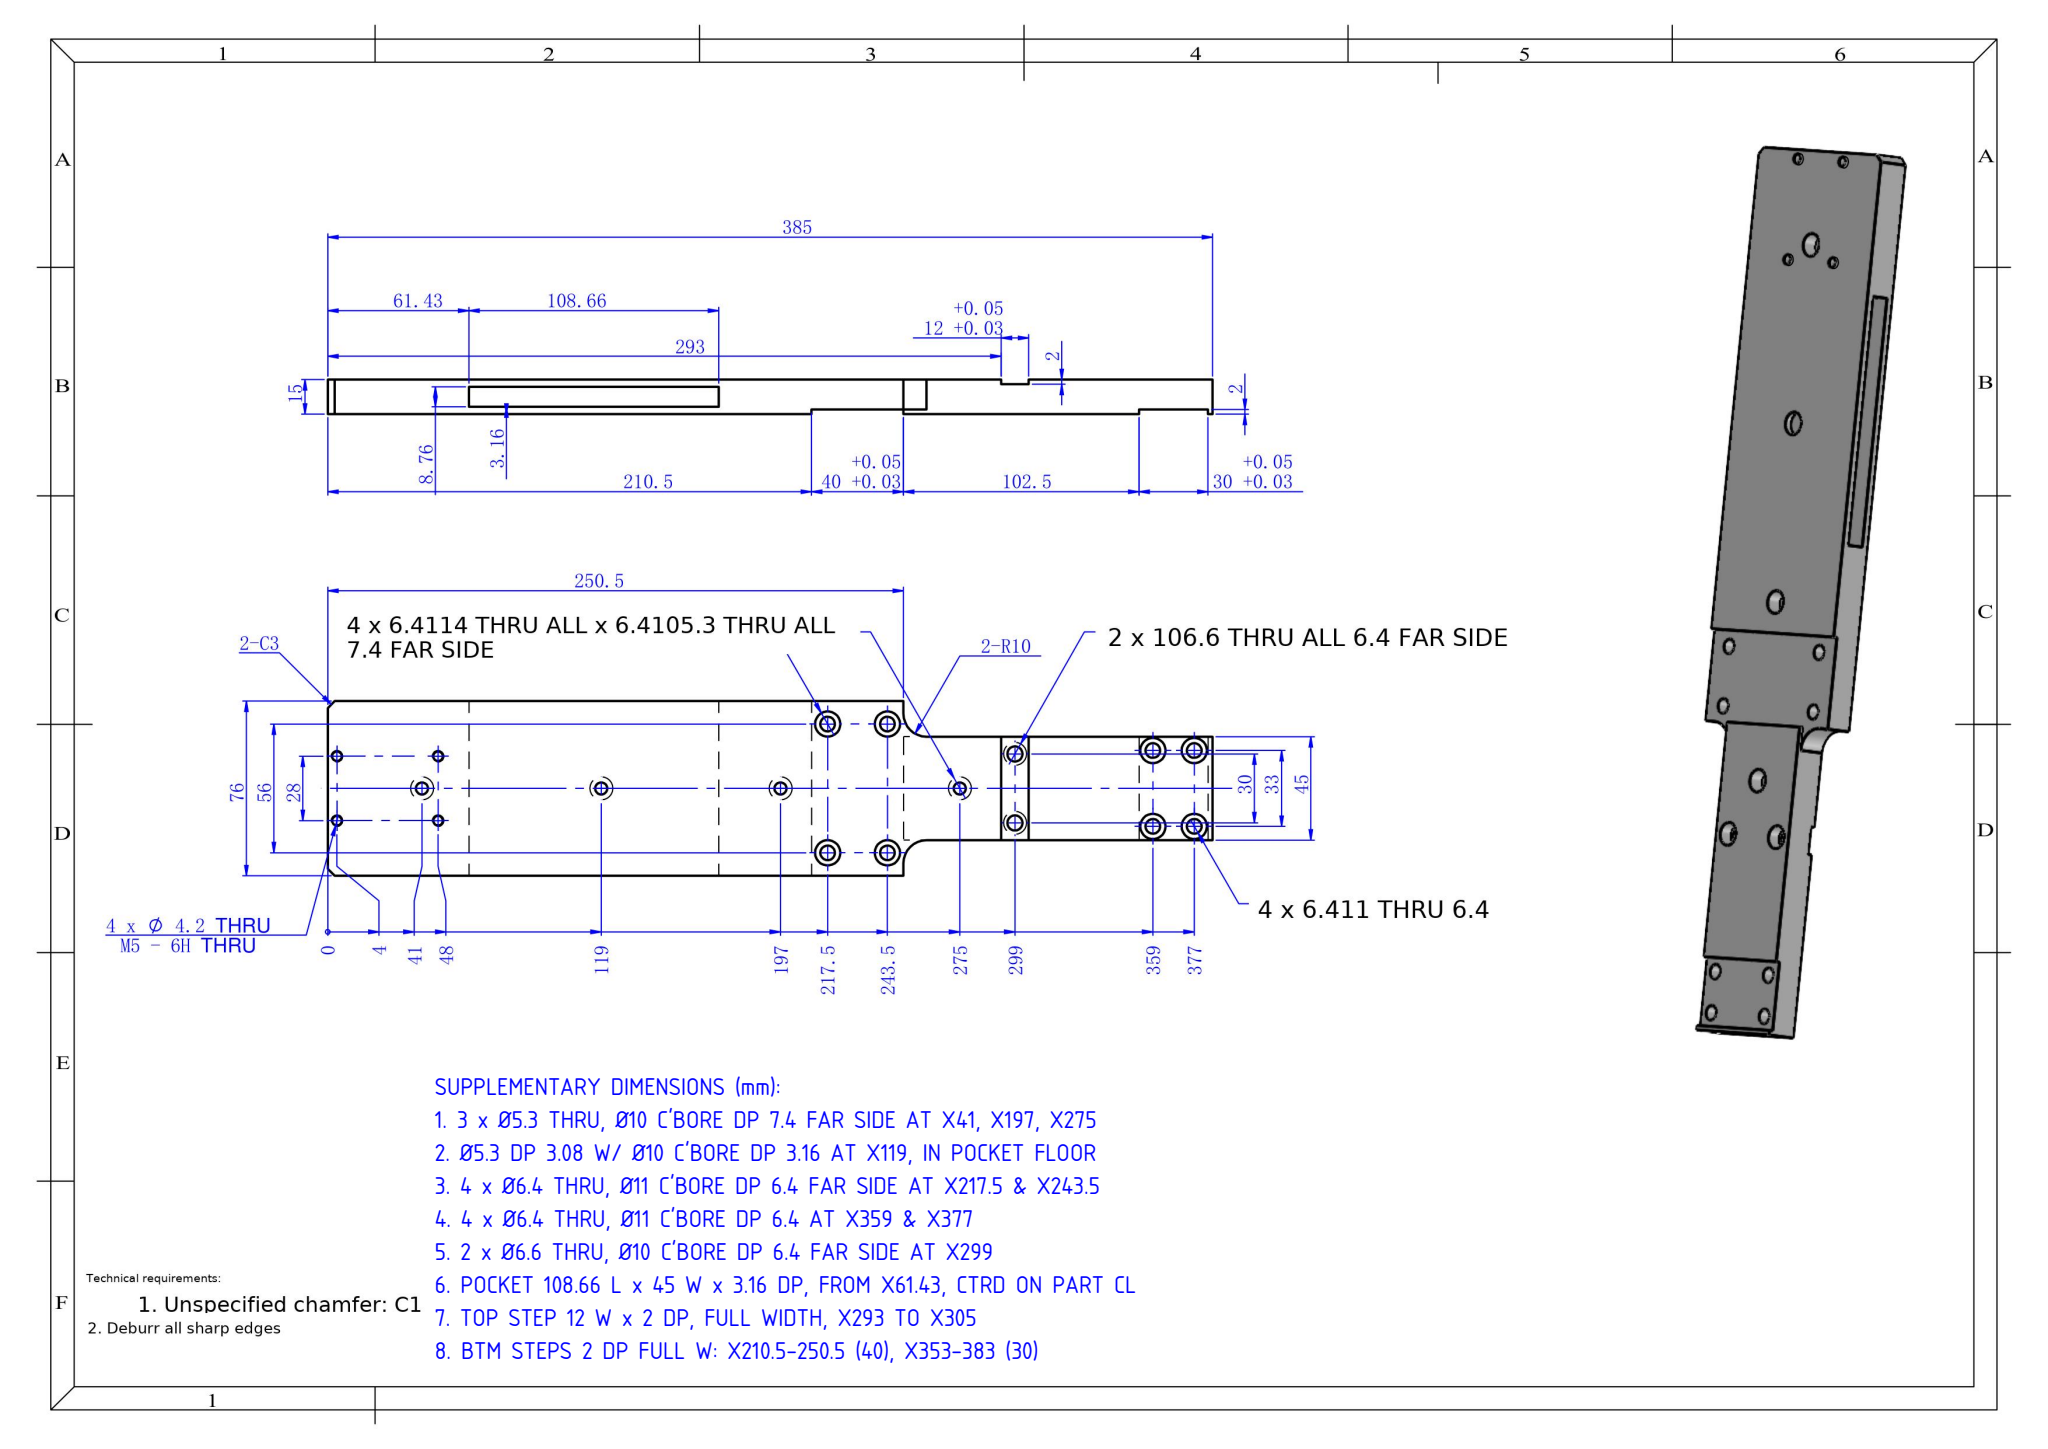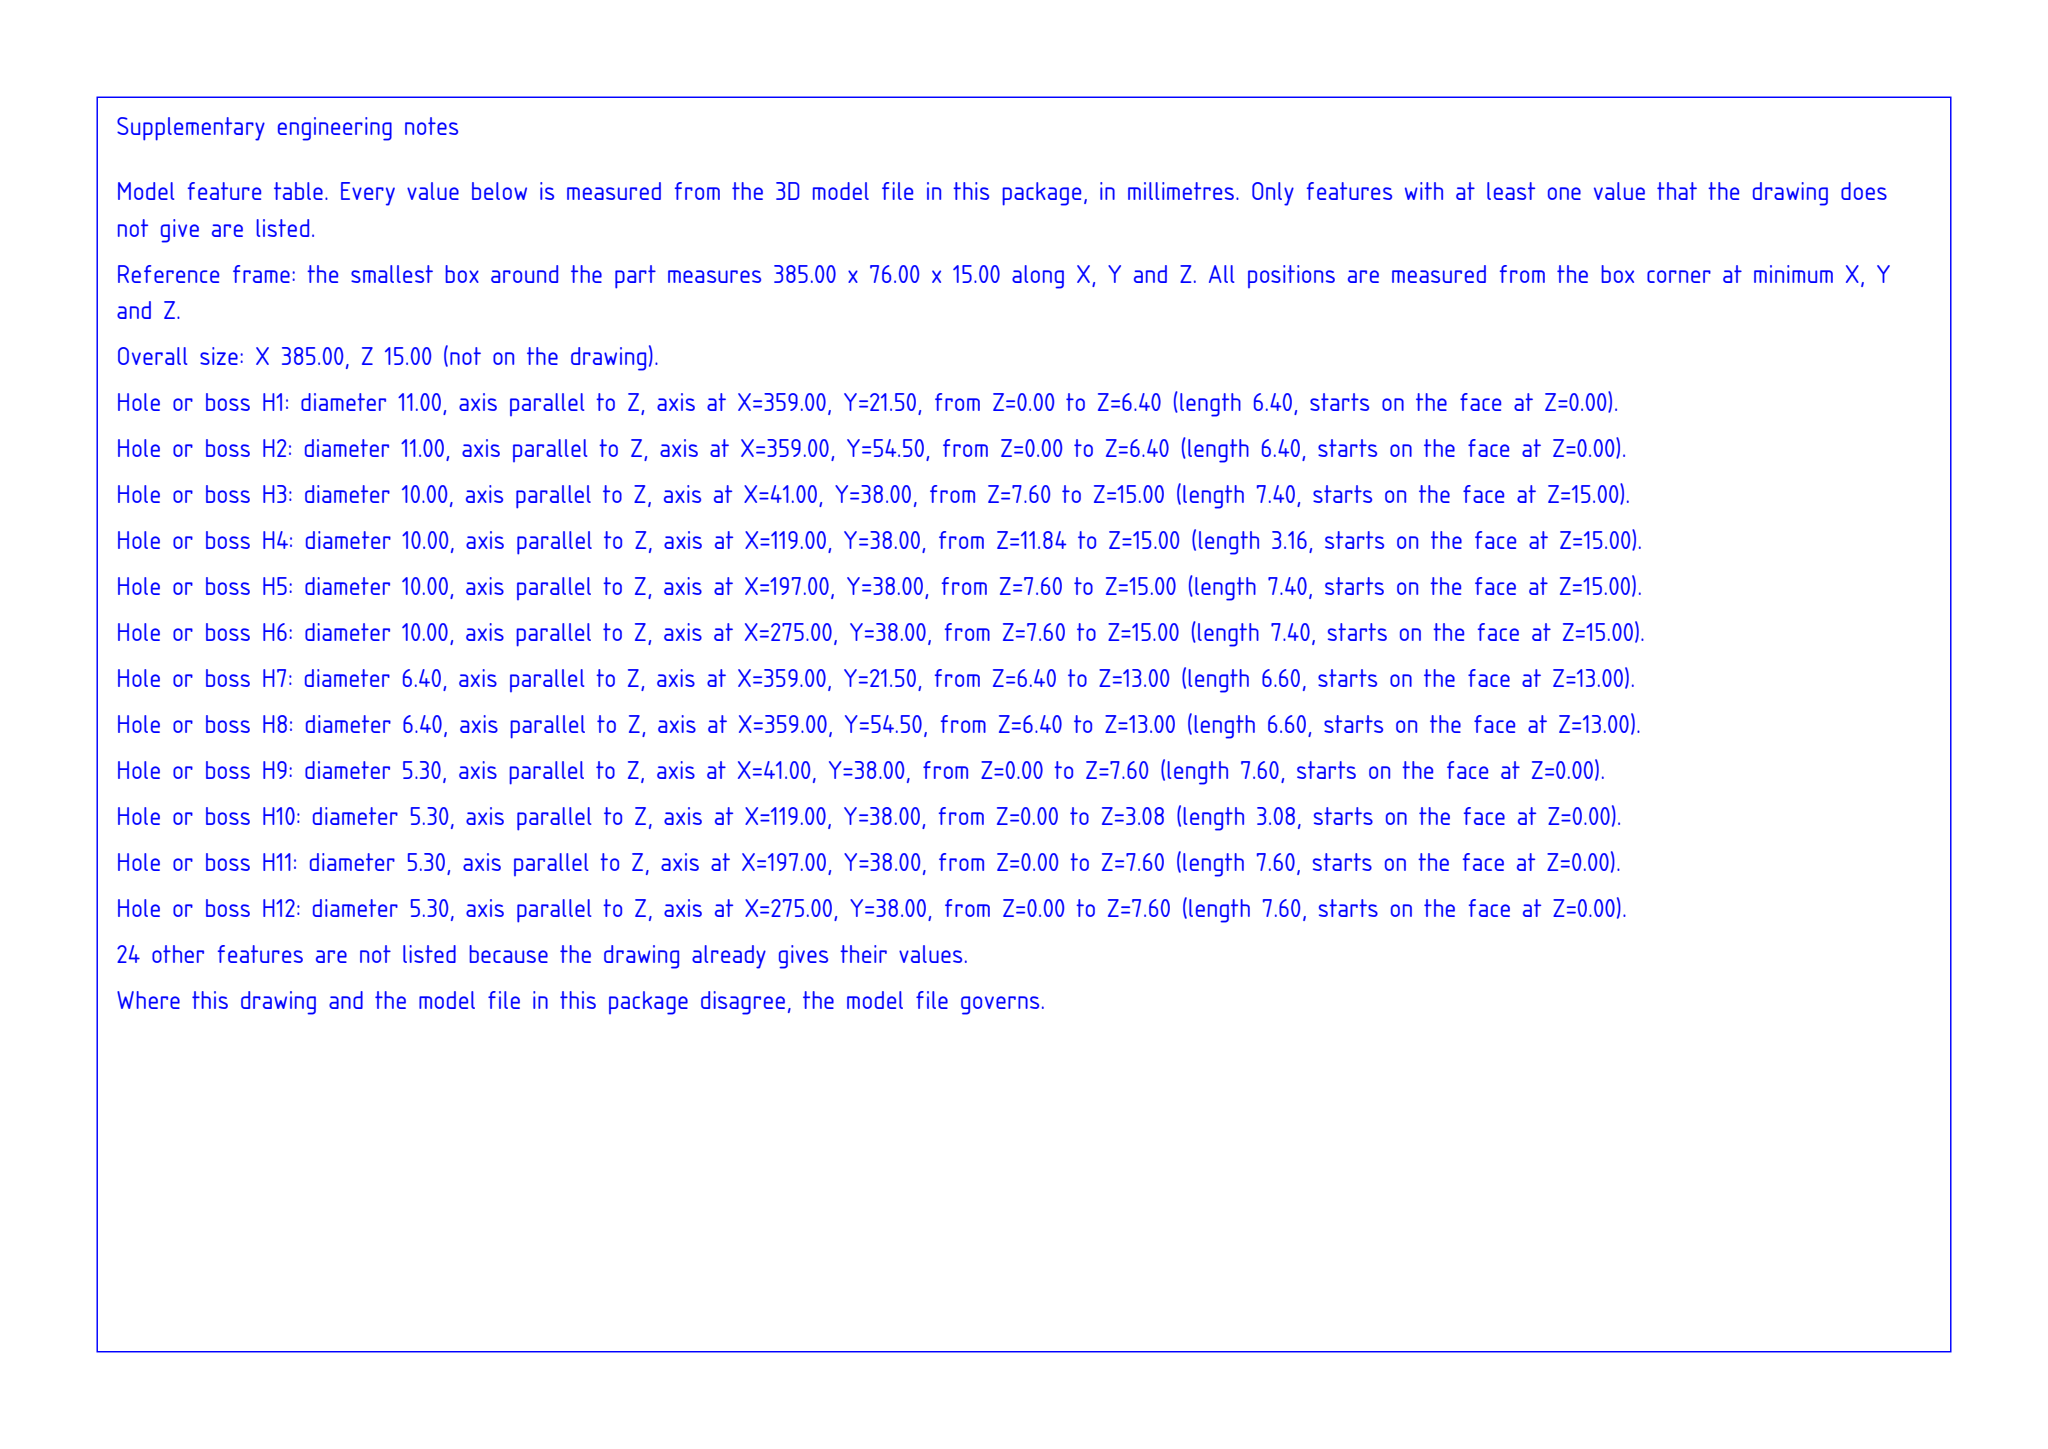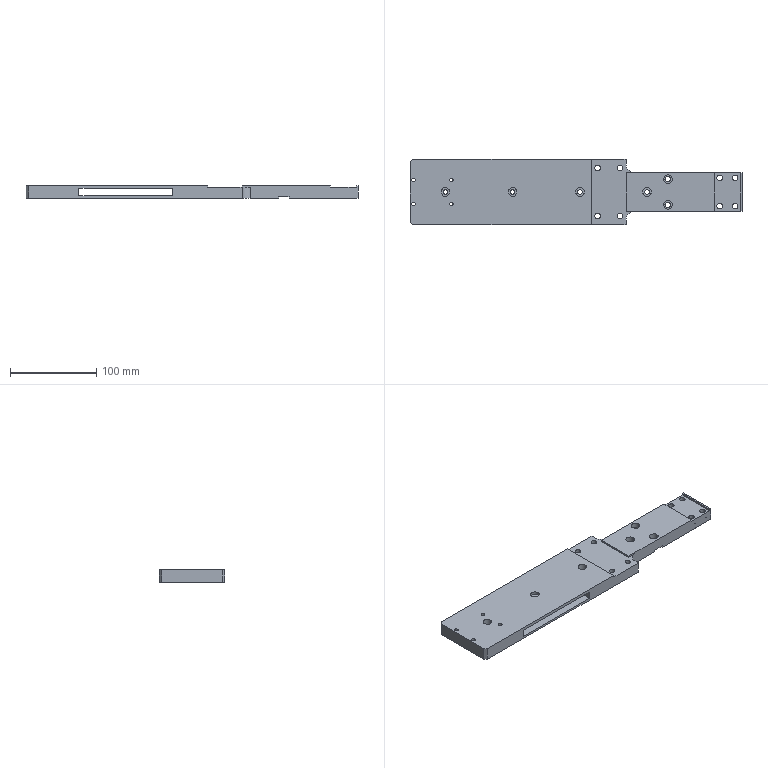Part | SolidWorks | mm | 1 solid | 107 faces | box 385 x 76 x 15 mm | volume 283123 mm3 | cylinder 66 | plane 41 | commonest cylinder face diameters 11 x16 6.4 x16 10 x12 4.2 x8 5.3 x8 6.6 x4 20 x2
build123d program:
from build123d import *

# Parameters (mm, degrees)
SKETCH1_W                                       = 385
SKETCH1_H                                       = 76
BOSS_EXTRUDE1_DEPTH                             = 15
SKETCH10_W                                      = 30
SKETCH10_H                                      = 2
SKETCH10_W_2                                    = 40
CUT_EXTRUDE5_DEPTH                              = 320.688
SKETCH12_W                                      = 134.5
SKETCH12_H                                      = 15.5
CUT_EXTRUDE10_DEPTH                             = 317.416
FILLET1_R                                       = 10
M6_HEX_SOCKET_HEAD_CAP_SCREW_CBORE1_D           = 6.4
M6_HEX_SOCKET_HEAD_CAP_SCREW_CBORE1_CBORE_D     = 11
M6_HEX_SOCKET_HEAD_CAP_SCREW_CBORE1_CBORE_DEPTH = 6.4
M6_HEX_SOCKET_HEAD_CAP_SCREW_CBORE2_D           = 6.4
M6_HEX_SOCKET_HEAD_CAP_SCREW_CBORE2_CBORE_D     = 11
M6_HEX_SOCKET_HEAD_CAP_SCREW_CBORE2_CBORE_DEPTH = 6.4
SKETCH17_W                                      = 12
SKETCH17_H                                      = 2
CUT_EXTRUDE11_DEPTH                             = 317.362
M5_HEX_SOCKET_HEAD_CAP_SCREW_CBORE1_D           = 5.3
M5_HEX_SOCKET_HEAD_CAP_SCREW_CBORE1_CBORE_D     = 10
M5_HEX_SOCKET_HEAD_CAP_SCREW_CBORE1_CBORE_DEPTH = 7.4
M5_TAPPED_HOLE1_D                               = 4.2
M6_HEX_SOCKET_HEAD_CAP_SCREW_CBORE3_D           = 6.6
M6_HEX_SOCKET_HEAD_CAP_SCREW_CBORE3_CBORE_D     = 10
M6_HEX_SOCKET_HEAD_CAP_SCREW_CBORE3_CBORE_DEPTH = 6.4
CHAMFER1_SIZE                                   = 3
SKETCH28_W                                      = 108.663
SKETCH28_H                                      = 8.765
CUT_EXTRUDE12_DEPTH                             = 133


with BuildPart() as part:
    # Sketch1 → Boss-Extrude1 (new body)
    with BuildSketch(Plane.XY):
        with Locations((117.661, 22.784)):
            Rectangle(SKETCH1_W, SKETCH1_H)
    extrude(amount=BOSS_EXTRUDE1_DEPTH)

    # Sketch10 → Cut-Extrude5 (cut, through all)
    with BuildSketch(Plane(origin=(0, 60.784, 0), x_dir=(1, 0, 0), z_dir=(0, 1, 0))):
        with Locations((293.161, -14)):
            Rectangle(SKETCH10_W, SKETCH10_H)
        with Locations((155.661, -14)):
            Rectangle(SKETCH10_W_2, SKETCH10_H)
    extrude(amount=-CUT_EXTRUDE5_DEPTH, mode=Mode.SUBTRACT)

    # Sketch12 → Cut-Extrude10 (cut, through all)
    with BuildSketch(Plane.XY.offset(15)):
        with Locations((242.911, 53.034)):
            Rectangle(SKETCH12_W, SKETCH12_H)
        with Locations((242.911, -7.466)):
            Rectangle(SKETCH12_W, SKETCH12_H)
    extrude(amount=-CUT_EXTRUDE10_DEPTH, mode=Mode.SUBTRACT)

    # Fillet1
    fillet1_edges = [part.edges().sort_by_distance(p)[0] for p in [
        (175.661, 45.284, 6.5),
        (175.661, 0.2842, 6.5),
    ]]
    fillet(fillet1_edges, radius=FILLET1_R)

    # M6 Hex Socket Head Cap Screw CBORE1 (through all)
    with Locations(Plane(origin=(0, 0, 0), x_dir=(-1, 0, 0), z_dir=(0, 0, -1))):
        with Locations((-284.161, 39.284), (-284.161, 6.284), (-302.161, 6.284), (-302.161, 39.284)):
            CounterBoreHole(M6_HEX_SOCKET_HEAD_CAP_SCREW_CBORE1_D / 2, M6_HEX_SOCKET_HEAD_CAP_SCREW_CBORE1_CBORE_D / 2, M6_HEX_SOCKET_HEAD_CAP_SCREW_CBORE1_CBORE_DEPTH)

    # M6 Hex Socket Head Cap Screw CBORE2 (through all)
    with Locations(Plane(origin=(0, 0, 0), x_dir=(-1, 0, 0), z_dir=(0, 0, -1))):
        with Locations((-142.661, 50.784), (-142.661, -5.216), (-168.661, -5.216), (-168.661, 50.784)):
            CounterBoreHole(M6_HEX_SOCKET_HEAD_CAP_SCREW_CBORE2_D / 2, M6_HEX_SOCKET_HEAD_CAP_SCREW_CBORE2_CBORE_D / 2, M6_HEX_SOCKET_HEAD_CAP_SCREW_CBORE2_CBORE_DEPTH)

    # Sketch17 → Cut-Extrude11 (cut, through all)
    with BuildSketch(Plane(origin=(0, 45.284, 0), x_dir=(1, 0, 0), z_dir=(0, 1, 0))):
        with Locations((224.161, -1)):
            Rectangle(SKETCH17_W, SKETCH17_H)
    extrude(amount=-CUT_EXTRUDE11_DEPTH, mode=Mode.SUBTRACT)

    # M5 Hex Socket Head Cap Screw CBORE1 (through all)
    with Locations(Plane.XY.offset(15)):
        with Locations((200.161, 22.784), (122.161, 22.784), (44.161, 22.784), (-33.839, 22.784)):
            CounterBoreHole(M5_HEX_SOCKET_HEAD_CAP_SCREW_CBORE1_D / 2, M5_HEX_SOCKET_HEAD_CAP_SCREW_CBORE1_CBORE_D / 2, M5_HEX_SOCKET_HEAD_CAP_SCREW_CBORE1_CBORE_DEPTH)

    # M5 Tapped Hole1 (through all)
    with Locations(Plane.XY.offset(15)):
        with Locations((-70.839, 8.784), (-70.839, 36.784), (-26.839, 36.784), (-26.839, 8.784)):
            Hole(M5_TAPPED_HOLE1_D / 2)

    # M6 Hex Socket Head Cap Screw CBORE3 (through all)
    with Locations(Plane.XY.offset(15)):
        with Locations((224.161, 37.784), (224.161, 7.784)):
            CounterBoreHole(M6_HEX_SOCKET_HEAD_CAP_SCREW_CBORE3_D / 2, M6_HEX_SOCKET_HEAD_CAP_SCREW_CBORE3_CBORE_D / 2, M6_HEX_SOCKET_HEAD_CAP_SCREW_CBORE3_CBORE_DEPTH)

    # Chamfer1
    chamfer1_edges = [part.edges().sort_by_distance(p)[0] for p in [
        (-74.839, 60.784, 7.5),
        (-74.839, -15.216, 7.5),
    ]]
    chamfer(chamfer1_edges, length=CHAMFER1_SIZE)

    # Sketch28 → Cut-Extrude12 (cut)
    with BuildSketch(Plane(origin=(0, 60.784, 0), x_dir=(1, 0, 0), z_dir=(0, 1, 0))):
        with Locations((40.917, -7.459)):
            Rectangle(SKETCH28_W, SKETCH28_H)
    extrude(amount=-CUT_EXTRUDE12_DEPTH, mode=Mode.SUBTRACT)


solid = part.part